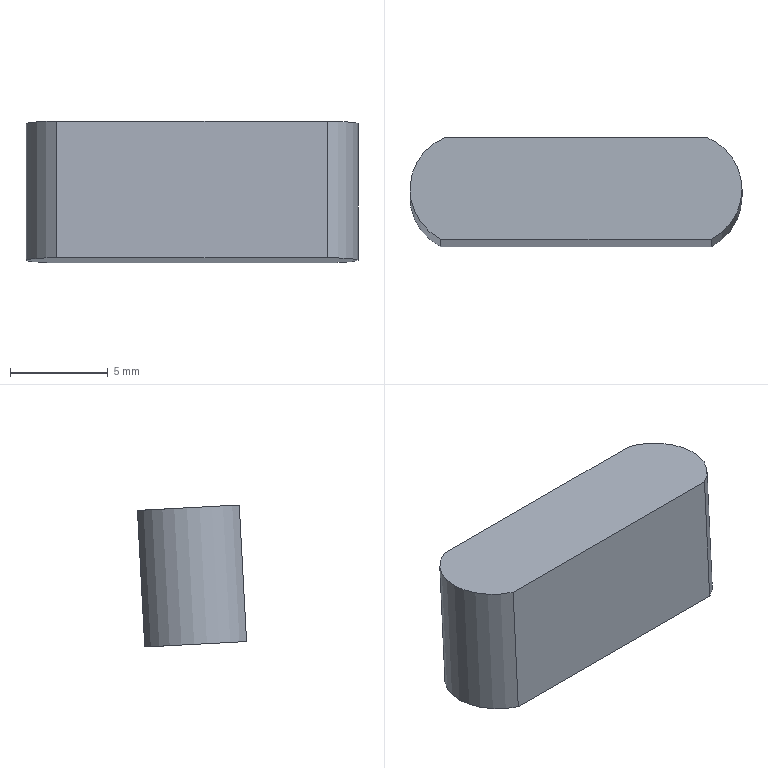Component | SolidWorks | ParallelKey5x5x25-1 | 1 solid | 7 faces | box 17 x 5.59 x 7.27 mm | volume 587 mm3 | plane 4 | cylinder 3 | commonest cylinder face diameters 5.732 x3
build123d program:
from build123d import *

# Parameters (mm, degrees)
BOSS_EXTRUDE1_DEPTH     = 7
CUT_EXTRUDE1_DEPTH      = 268.356
CUT_EXTRUDE1_DEPTH_BACK = 268.356


with BuildPart() as part:
    # Sketch1 → Boss-Extrude1 (new body)
    with BuildSketch(Plane.XY):
        Polygon((-256.993, 2.611), (-262.252, 2.611), (-267.252, 2.611), (-267.252, -2.611), (-262.252, -2.611), (-256.993, -2.611), (-250.252, -2.611), (-250.252, 2.611), align=None)
    extrude(amount=BOSS_EXTRUDE1_DEPTH)

    # Sketch2 → Cut-Extrude1 (cut, two sides: drawn at the far end of the back side and taken through both)
    with BuildSketch(Plane.XY.offset(7).offset(-CUT_EXTRUDE1_DEPTH_BACK)):
        with BuildLine():
            Line((-267.252, 2.611), (-267.252, -0.05342))
            ThreePointArc((-267.252, -0.05342), (-266.757, 1.557), (-265.442, 2.611))
            Line((-265.442, 2.611), (-267.252, 2.611))
        make_face()
        with BuildLine():
            Line((-267.252, -0.05342), (-267.252, -2.611))
            Line((-267.252, -2.611), (-265.68, -2.611))
            ThreePointArc((-265.68, -2.611), (-266.828, -1.554), (-267.252, -0.05342))
        make_face()
        with BuildLine():
            ThreePointArc((-252.062, 2.611), (-250.747, 1.557), (-250.252, -0.05342))
            Line((-250.252, -0.05342), (-250.252, 2.611))
            Line((-250.252, 2.611), (-252.062, 2.611))
        make_face()
        with BuildLine():
            ThreePointArc((-250.252, -0.05342), (-250.676, -1.554), (-251.824, -2.611))
            Line((-251.824, -2.611), (-250.252, -2.611))
            Line((-250.252, -2.611), (-250.252, -0.05342))
        make_face()
    extrude(amount=CUT_EXTRUDE1_DEPTH + CUT_EXTRUDE1_DEPTH_BACK, mode=Mode.SUBTRACT)


solid = part.part

# Placed as in the assembly
solid = solid.moved(Location((-14.748, 60.343, 2.317), (-3.057, 0, 0)))
STEP:
#1=COLOUR_RGB('',0.7922,0.8196,0.9333);
#2=FILL_AREA_STYLE_COLOUR('',#1);
#3=FILL_AREA_STYLE('',(#2));
#4=SURFACE_STYLE_FILL_AREA(#3);
#5=SURFACE_SIDE_STYLE('',(#4));
#6=SURFACE_STYLE_USAGE(.BOTH.,#5);
#7=PRESENTATION_STYLE_ASSIGNMENT((#6));
#8=CARTESIAN_POINT('',(-10.433,2.374,0.09134));
#9=VERTEX_POINT('',#8);
#10=CARTESIAN_POINT('',(-10.495,2.273,0.09671));
#11=VERTEX_POINT('',#10);
#12=CARTESIAN_POINT('',(-10.546,2.374,0.09134));
#13=DIRECTION('',(0.,-0.05333,-0.9986));
#14=DIRECTION('',(1.,0.,0.));
#15=AXIS2_PLACEMENT_3D('',#12,#13,#14);
#16=CIRCLE('',#15,0.1128);
#17=EDGE_CURVE('',#9,#11,#16,.T.);
#18=ORIENTED_EDGE('',*,*,#17,.F.);
#19=CARTESIAN_POINT('',(-10.433,2.388,0.3665));
#20=VERTEX_POINT('',#19);
#21=CARTESIAN_POINT('',(-10.433,2.374,0.09134));
#22=DIRECTION('',(-0.,0.05333,0.9986));
#23=VECTOR('',#22,39.37);
#24=LINE('',#21,#23);
#25=EDGE_CURVE('',#9,#20,#24,.T.);
#26=ORIENTED_EDGE('',*,*,#25,.T.);
#27=CARTESIAN_POINT('',(-10.495,2.288,0.3719));
#28=VERTEX_POINT('',#27);
#29=CARTESIAN_POINT('',(-10.546,2.388,0.3665));
#30=DIRECTION('',(0.,-0.05333,-0.9986));
#31=DIRECTION('',(1.,0.,0.));
#32=AXIS2_PLACEMENT_3D('',#29,#30,#31);
#33=CIRCLE('',#32,0.1128);
#34=EDGE_CURVE('',#20,#28,#33,.T.);
#35=ORIENTED_EDGE('',*,*,#34,.T.);
#36=CARTESIAN_POINT('',(-10.495,2.273,0.09671));
#37=DIRECTION('',(-0.,0.05333,0.9986));
#38=VECTOR('',#37,39.37);
#39=LINE('',#36,#38);
#40=EDGE_CURVE('',#11,#28,#39,.T.);
#41=ORIENTED_EDGE('',*,*,#40,.F.);
#42=EDGE_LOOP('',(#18,#26,#35,#41));
#43=FACE_OUTER_BOUND('',#42,.T.);
#44=CARTESIAN_POINT('',(-10.546,2.374,0.09134));
#45=DIRECTION('',(-0.,0.05333,0.9986));
#46=DIRECTION('',(1.,0.,0.));
#47=AXIS2_PLACEMENT_3D('',#44,#45,#46);
#48=CYLINDRICAL_SURFACE('',#47,0.1128);
#49=ADVANCED_FACE('',(#43),#48,.T.);
#50=CARTESIAN_POINT('',(-11.031,2.493,0.3609));
#51=VERTEX_POINT('',#50);
#52=CARTESIAN_POINT('',(-11.04,2.288,0.3719));
#53=VERTEX_POINT('',#52);
#54=CARTESIAN_POINT('',(-10.99,2.388,0.3665));
#55=DIRECTION('',(-0.,0.05333,0.9986));
#56=DIRECTION('',(1.,0.,0.));
#57=AXIS2_PLACEMENT_3D('',#54,#55,#56);
#58=CIRCLE('',#57,0.1128);
#59=EDGE_CURVE('',#51,#53,#58,.T.);
#60=ORIENTED_EDGE('',*,*,#59,.T.);
#61=CARTESIAN_POINT('',(-0.5806,2.288,0.3719));
#62=DIRECTION('',(1.,-0.,0.));
#63=VECTOR('',#62,39.37);
#64=LINE('',#61,#63);
#65=EDGE_CURVE('',#53,#28,#64,.T.);
#66=ORIENTED_EDGE('',*,*,#65,.T.);
#67=ORIENTED_EDGE('',*,*,#34,.F.);
#68=CARTESIAN_POINT('',(-10.504,2.493,0.3609));
#69=VERTEX_POINT('',#68);
#70=CARTESIAN_POINT('',(-10.546,2.388,0.3665));
#71=DIRECTION('',(0.,-0.05333,-0.9986));
#72=DIRECTION('',(1.,0.,-0.));
#73=AXIS2_PLACEMENT_3D('',#70,#71,#72);
#74=CIRCLE('',#73,0.1128);
#75=EDGE_CURVE('',#69,#20,#74,.T.);
#76=ORIENTED_EDGE('',*,*,#75,.F.);
#77=CARTESIAN_POINT('',(-0.5806,2.493,0.3609));
#78=DIRECTION('',(-1.,0.,-0.));
#79=VECTOR('',#78,39.37);
#80=LINE('',#77,#79);
#81=EDGE_CURVE('',#69,#51,#80,.T.);
#82=ORIENTED_EDGE('',*,*,#81,.T.);
#83=EDGE_LOOP('',(#60,#66,#67,#76,#82));
#84=FACE_OUTER_BOUND('',#83,.T.);
#85=CARTESIAN_POINT('',(-0.5806,2.39,0.3664));
#86=DIRECTION('',(-0.,0.05333,0.9986));
#87=DIRECTION('',(1.,-0.,0.));
#88=AXIS2_PLACEMENT_3D('',#85,#86,#87);
#89=PLANE('',#88);
#90=ADVANCED_FACE('',(#84),#89,.T.);
#91=CARTESIAN_POINT('',(-11.04,2.273,0.09671));
#92=VERTEX_POINT('',#91);
#93=CARTESIAN_POINT('',(-0.5806,2.273,0.09671));
#94=DIRECTION('',(1.,-0.,0.));
#95=VECTOR('',#94,39.37);
#96=LINE('',#93,#95);
#97=EDGE_CURVE('',#92,#11,#96,.T.);
#98=ORIENTED_EDGE('',*,*,#97,.F.);
#99=CARTESIAN_POINT('',(-11.031,2.478,0.08575));
#100=VERTEX_POINT('',#99);
#101=CARTESIAN_POINT('',(-10.99,2.374,0.09134));
#102=DIRECTION('',(-0.,0.05333,0.9986));
#103=DIRECTION('',(1.,0.,0.));
#104=AXIS2_PLACEMENT_3D('',#101,#102,#103);
#105=CIRCLE('',#104,0.1128);
#106=EDGE_CURVE('',#100,#92,#105,.T.);
#107=ORIENTED_EDGE('',*,*,#106,.F.);
#108=CARTESIAN_POINT('',(-10.504,2.478,0.08575));
#109=VERTEX_POINT('',#108);
#110=CARTESIAN_POINT('',(-0.5806,2.478,0.08575));
#111=DIRECTION('',(-1.,0.,-0.));
#112=VECTOR('',#111,39.37);
#113=LINE('',#110,#112);
#114=EDGE_CURVE('',#109,#100,#113,.T.);
#115=ORIENTED_EDGE('',*,*,#114,.F.);
#116=CARTESIAN_POINT('',(-10.546,2.374,0.09134));
#117=DIRECTION('',(0.,-0.05333,-0.9986));
#118=DIRECTION('',(1.,0.,-0.));
#119=AXIS2_PLACEMENT_3D('',#116,#117,#118);
#120=CIRCLE('',#119,0.1128);
#121=EDGE_CURVE('',#109,#9,#120,.T.);
#122=ORIENTED_EDGE('',*,*,#121,.T.);
#123=ORIENTED_EDGE('',*,*,#17,.T.);
#124=EDGE_LOOP('',(#98,#107,#115,#122,#123));
#125=FACE_OUTER_BOUND('',#124,.T.);
#126=CARTESIAN_POINT('',(-0.5806,2.376,0.09123));
#127=DIRECTION('',(-0.,0.05333,0.9986));
#128=DIRECTION('',(1.,-0.,0.));
#129=AXIS2_PLACEMENT_3D('',#126,#127,#128);
#130=PLANE('',#129);
#131=ADVANCED_FACE('',(#125),#130,.F.);
#132=CARTESIAN_POINT('',(-11.04,2.273,0.09671));
#133=DIRECTION('',(-0.,0.05333,0.9986));
#134=VECTOR('',#133,39.37);
#135=LINE('',#132,#134);
#136=EDGE_CURVE('',#92,#53,#135,.T.);
#137=ORIENTED_EDGE('',*,*,#136,.F.);
#138=ORIENTED_EDGE('',*,*,#97,.T.);
#139=ORIENTED_EDGE('',*,*,#40,.T.);
#140=ORIENTED_EDGE('',*,*,#65,.F.);
#141=EDGE_LOOP('',(#137,#138,#139,#140));
#142=FACE_OUTER_BOUND('',#141,.T.);
#143=CARTESIAN_POINT('',(-0.5806,2.288,0.3719));
#144=DIRECTION('',(0.,0.9986,-0.05333));
#145=DIRECTION('',(-1.,0.,-0.));
#146=AXIS2_PLACEMENT_3D('',#143,#144,#145);
#147=PLANE('',#146);
#148=ADVANCED_FACE('',(#142),#147,.F.);
#149=ORIENTED_EDGE('',*,*,#81,.F.);
#150=CARTESIAN_POINT('',(-10.504,2.478,0.08575));
#151=DIRECTION('',(-0.,0.05333,0.9986));
#152=VECTOR('',#151,39.37);
#153=LINE('',#150,#152);
#154=EDGE_CURVE('',#109,#69,#153,.T.);
#155=ORIENTED_EDGE('',*,*,#154,.F.);
#156=ORIENTED_EDGE('',*,*,#114,.T.);
#157=CARTESIAN_POINT('',(-11.031,2.478,0.08575));
#158=DIRECTION('',(-0.,0.05333,0.9986));
#159=VECTOR('',#158,39.37);
#160=LINE('',#157,#159);
#161=EDGE_CURVE('',#100,#51,#160,.T.);
#162=ORIENTED_EDGE('',*,*,#161,.T.);
#163=EDGE_LOOP('',(#149,#155,#156,#162));
#164=FACE_OUTER_BOUND('',#163,.T.);
#165=CARTESIAN_POINT('',(-0.5806,2.493,0.3609));
#166=DIRECTION('',(-0.,-0.9986,0.05333));
#167=DIRECTION('',(1.,-0.,0.));
#168=AXIS2_PLACEMENT_3D('',#165,#166,#167);
#169=PLANE('',#168);
#170=ADVANCED_FACE('',(#164),#169,.F.);
#171=ORIENTED_EDGE('',*,*,#25,.F.);
#172=ORIENTED_EDGE('',*,*,#121,.F.);
#173=ORIENTED_EDGE('',*,*,#154,.T.);
#174=ORIENTED_EDGE('',*,*,#75,.T.);
#175=EDGE_LOOP('',(#171,#172,#173,#174));
#176=FACE_OUTER_BOUND('',#175,.T.);
#177=CARTESIAN_POINT('',(-10.546,2.374,0.09134));
#178=DIRECTION('',(-0.,0.05333,0.9986));
#179=DIRECTION('',(1.,0.,0.));
#180=AXIS2_PLACEMENT_3D('',#177,#178,#179);
#181=CYLINDRICAL_SURFACE('',#180,0.1128);
#182=ADVANCED_FACE('',(#176),#181,.T.);
#183=ORIENTED_EDGE('',*,*,#161,.F.);
#184=ORIENTED_EDGE('',*,*,#106,.T.);
#185=ORIENTED_EDGE('',*,*,#136,.T.);
#186=ORIENTED_EDGE('',*,*,#59,.F.);
#187=EDGE_LOOP('',(#183,#184,#185,#186));
#188=FACE_OUTER_BOUND('',#187,.T.);
#189=CARTESIAN_POINT('',(-10.99,2.374,0.09134));
#190=DIRECTION('',(-0.,0.05333,0.9986));
#191=DIRECTION('',(1.,0.,0.));
#192=AXIS2_PLACEMENT_3D('',#189,#190,#191);
#193=CYLINDRICAL_SURFACE('',#192,0.1128);
#194=ADVANCED_FACE('',(#188),#193,.T.);
#195=CLOSED_SHELL('',(#49,#90,#131,#148,#170,#182,#194));
#196=MANIFOLD_SOLID_BREP('',#195);
#197=STYLED_ITEM('',(#7),#196);
#198=PRESENTATION_LAYER_ASSIGNMENT('','',(#197));
#199=(LENGTH_UNIT()NAMED_UNIT(*)SI_UNIT($,.METRE.));
#200=LENGTH_MEASURE_WITH_UNIT(LENGTH_MEASURE(0.0254),#199);
#201=DIMENSIONAL_EXPONENTS(1.,0.,0.,0.,0.,0.,0.);
#202=(CONVERSION_BASED_UNIT('',#200)LENGTH_UNIT()NAMED_UNIT(#201));
#203=UNCERTAINTY_MEASURE_WITH_UNIT(LENGTH_MEASURE(0.00001),#202,'','');
#204=(NAMED_UNIT(*)PLANE_ANGLE_UNIT()SI_UNIT($,.RADIAN.));
#205=(NAMED_UNIT(*)SI_UNIT($,.STERADIAN.)SOLID_ANGLE_UNIT());
#206=(GEOMETRIC_REPRESENTATION_CONTEXT(3)GLOBAL_UNCERTAINTY_ASSIGNED_CONTEXT((#203))GLOBAL_UNIT_ASSIGNED_CONTEXT((#202,#204,#205))REPRESENTATION_CONTEXT('',''));
#207=MECHANICAL_DESIGN_GEOMETRIC_PRESENTATION_REPRESENTATION('',(#197),#206);
#208=CARTESIAN_POINT('',(0.,0.,0.));
#209=DIRECTION('',(0.,0.,1.));
#210=DIRECTION('',(1.,0.,0.));
#211=AXIS2_PLACEMENT_3D('',#208,#209,#210);
#212=(LENGTH_UNIT()NAMED_UNIT(*)SI_UNIT($,.METRE.));
#213=LENGTH_MEASURE_WITH_UNIT(LENGTH_MEASURE(0.0254),#212);
#214=DIMENSIONAL_EXPONENTS(1.,0.,0.,0.,0.,0.,0.);
#215=(CONVERSION_BASED_UNIT('',#213)LENGTH_UNIT()NAMED_UNIT(#214));
#216=UNCERTAINTY_MEASURE_WITH_UNIT(LENGTH_MEASURE(0.00001),#215,'','');
#217=(NAMED_UNIT(*)PLANE_ANGLE_UNIT()SI_UNIT($,.RADIAN.));
#218=(NAMED_UNIT(*)SI_UNIT($,.STERADIAN.)SOLID_ANGLE_UNIT());
#219=(GEOMETRIC_REPRESENTATION_CONTEXT(3)GLOBAL_UNCERTAINTY_ASSIGNED_CONTEXT((#216))GLOBAL_UNIT_ASSIGNED_CONTEXT((#215,#217,#218))REPRESENTATION_CONTEXT('',''));
#220=ADVANCED_BREP_SHAPE_REPRESENTATION('',(#196,#211),#219);